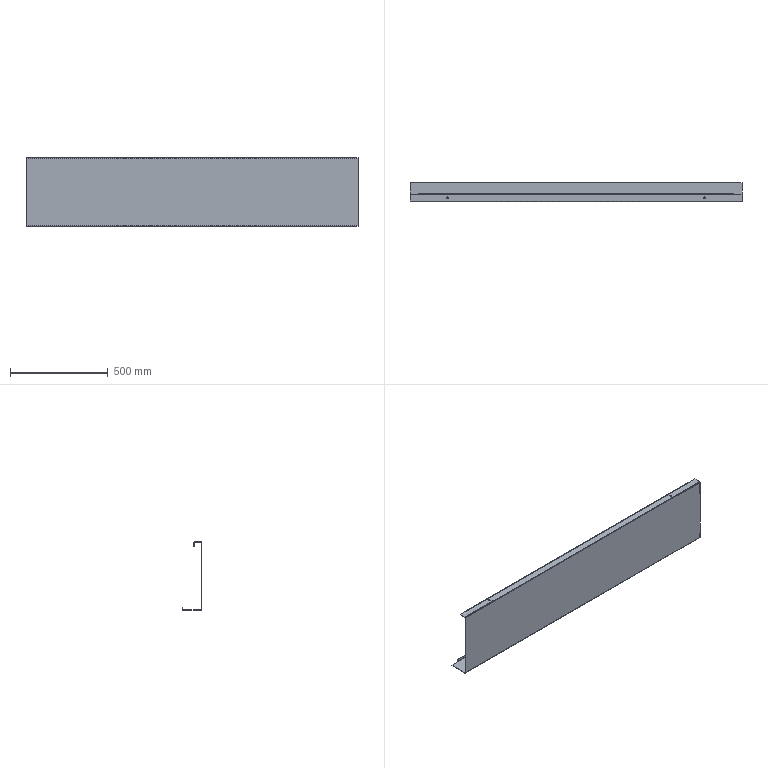Component | SolidWorks | LeftSidePlate-1 | 1 solid | 42 faces | volume 1756131 mm3 | plane 30 | cylinder 12 | commonest cylinder face diameters 8.5 x4 6 x4 2 x4